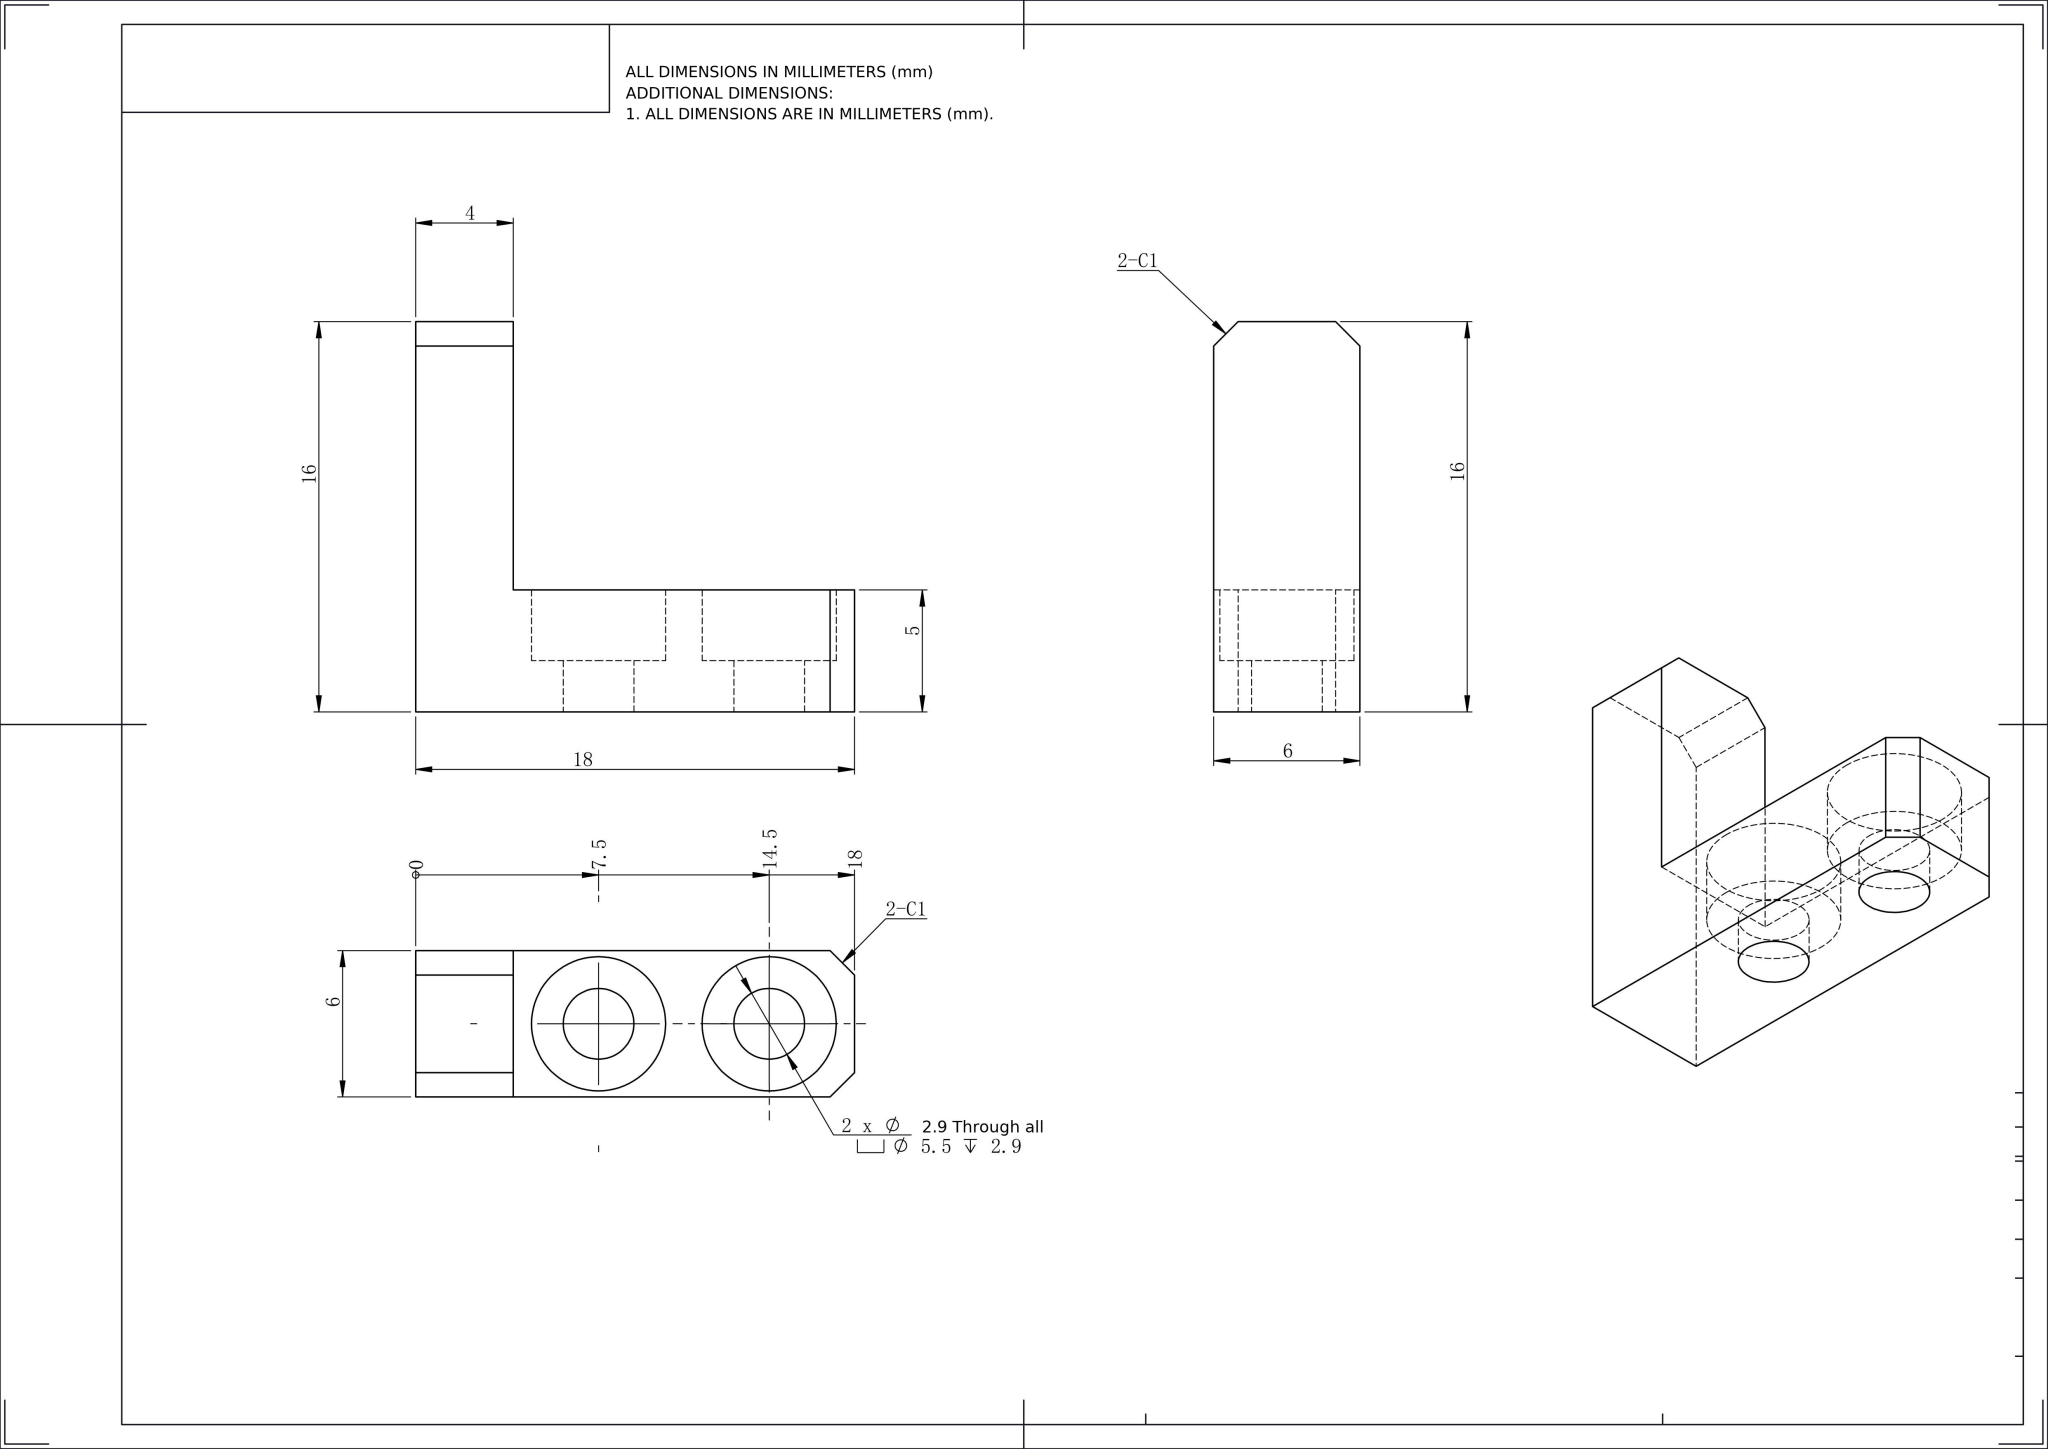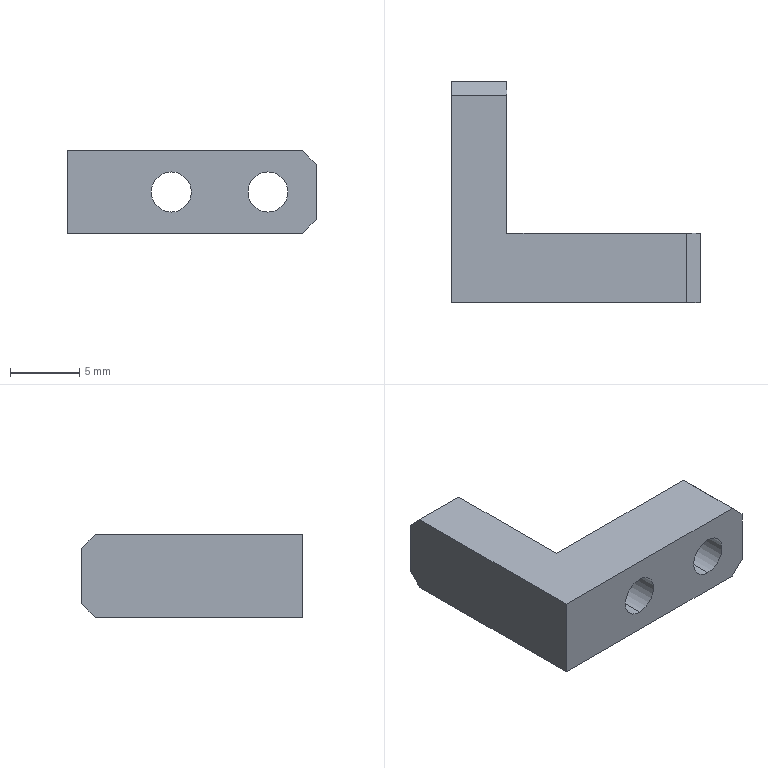Part | NX | mm | Chamfered Dual-Bore Clevis Block | 1 solid | 22 faces | box 18 x 16 x 6 mm | volume 629 mm3 | plane 14 | cylinder 8 | commonest cylinder face diameters 5.5 x4 2.9 x4
STEP:
#1=COLOUR_RGB('',0.7922,0.8196,0.9333);
#2=FILL_AREA_STYLE_COLOUR('',#1);
#3=FILL_AREA_STYLE('',(#2));
#4=SURFACE_STYLE_FILL_AREA(#3);
#5=SURFACE_SIDE_STYLE('',(#4));
#6=SURFACE_STYLE_USAGE(.BOTH.,#5);
#7=PRESENTATION_STYLE_ASSIGNMENT((#6));
#8=CARTESIAN_POINT('',(5.5,-5.9,-2.75));
#9=VERTEX_POINT('',#8);
#10=CARTESIAN_POINT('',(5.5,-5.9,2.75));
#11=VERTEX_POINT('',#10);
#12=CARTESIAN_POINT('',(5.5,-5.9,0.));
#13=DIRECTION('',(0.,1.,0.));
#14=DIRECTION('',(0.,0.,1.));
#15=AXIS2_PLACEMENT_3D('',#12,#13,#14);
#16=CIRCLE('',#15,2.75);
#17=EDGE_CURVE('',#9,#11,#16,.T.);
#18=ORIENTED_EDGE('',*,*,#17,.F.);
#19=CARTESIAN_POINT('',(5.5,-3.,-2.75));
#20=VERTEX_POINT('',#19);
#21=CARTESIAN_POINT('',(5.5,-3.,-2.75));
#22=DIRECTION('',(0.,1.,0.));
#23=VECTOR('',#22,1000.);
#24=LINE('',#21,#23);
#25=EDGE_CURVE('',#9,#20,#24,.T.);
#26=ORIENTED_EDGE('',*,*,#25,.T.);
#27=CARTESIAN_POINT('',(5.5,-3.,2.75));
#28=VERTEX_POINT('',#27);
#29=CARTESIAN_POINT('',(5.5,-3.,0.));
#30=DIRECTION('',(0.,1.,0.));
#31=DIRECTION('',(0.,0.,1.));
#32=AXIS2_PLACEMENT_3D('',#29,#30,#31);
#33=CIRCLE('',#32,2.75);
#34=EDGE_CURVE('',#20,#28,#33,.T.);
#35=ORIENTED_EDGE('',*,*,#34,.T.);
#36=CARTESIAN_POINT('',(5.5,-3.,2.75));
#37=DIRECTION('',(0.,1.,0.));
#38=VECTOR('',#37,1000.);
#39=LINE('',#36,#38);
#40=EDGE_CURVE('',#11,#28,#39,.T.);
#41=ORIENTED_EDGE('',*,*,#40,.F.);
#42=EDGE_LOOP('',(#18,#26,#35,#41));
#43=FACE_OUTER_BOUND('',#42,.T.);
#44=CARTESIAN_POINT('',(5.5,-3.,0.));
#45=DIRECTION('',(0.,1.,0.));
#46=DIRECTION('',(0.,0.,1.));
#47=AXIS2_PLACEMENT_3D('',#44,#45,#46);
#48=CYLINDRICAL_SURFACE('',#47,2.75);
#49=ADVANCED_FACE('',(#43),#48,.F.);
#50=CARTESIAN_POINT('',(5.5,-8.,-1.45));
#51=VERTEX_POINT('',#50);
#52=CARTESIAN_POINT('',(5.5,-8.,1.45));
#53=VERTEX_POINT('',#52);
#54=CARTESIAN_POINT('',(5.5,-8.,0.));
#55=DIRECTION('',(0.,1.,0.));
#56=DIRECTION('',(0.,0.,1.));
#57=AXIS2_PLACEMENT_3D('',#54,#55,#56);
#58=CIRCLE('',#57,1.45);
#59=EDGE_CURVE('',#51,#53,#58,.T.);
#60=ORIENTED_EDGE('',*,*,#59,.F.);
#61=CARTESIAN_POINT('',(5.5,-5.9,-1.45));
#62=VERTEX_POINT('',#61);
#63=CARTESIAN_POINT('',(5.5,-3.,-1.45));
#64=DIRECTION('',(0.,1.,0.));
#65=VECTOR('',#64,1000.);
#66=LINE('',#63,#65);
#67=EDGE_CURVE('',#51,#62,#66,.T.);
#68=ORIENTED_EDGE('',*,*,#67,.T.);
#69=CARTESIAN_POINT('',(5.5,-5.9,1.45));
#70=VERTEX_POINT('',#69);
#71=CARTESIAN_POINT('',(5.5,-5.9,0.));
#72=DIRECTION('',(0.,1.,0.));
#73=DIRECTION('',(0.,0.,1.));
#74=AXIS2_PLACEMENT_3D('',#71,#72,#73);
#75=CIRCLE('',#74,1.45);
#76=EDGE_CURVE('',#62,#70,#75,.T.);
#77=ORIENTED_EDGE('',*,*,#76,.T.);
#78=CARTESIAN_POINT('',(5.5,-3.,1.45));
#79=DIRECTION('',(0.,1.,0.));
#80=VECTOR('',#79,1000.);
#81=LINE('',#78,#80);
#82=EDGE_CURVE('',#53,#70,#81,.T.);
#83=ORIENTED_EDGE('',*,*,#82,.F.);
#84=EDGE_LOOP('',(#60,#68,#77,#83));
#85=FACE_OUTER_BOUND('',#84,.T.);
#86=CARTESIAN_POINT('',(5.5,-3.,0.));
#87=DIRECTION('',(0.,1.,0.));
#88=DIRECTION('',(0.,0.,1.));
#89=AXIS2_PLACEMENT_3D('',#86,#87,#88);
#90=CYLINDRICAL_SURFACE('',#89,1.45);
#91=ADVANCED_FACE('',(#85),#90,.F.);
#92=CARTESIAN_POINT('',(-1.5,-5.9,-2.75));
#93=VERTEX_POINT('',#92);
#94=CARTESIAN_POINT('',(-1.5,-5.9,2.75));
#95=VERTEX_POINT('',#94);
#96=CARTESIAN_POINT('',(-1.5,-5.9,0.));
#97=DIRECTION('',(0.,1.,0.));
#98=DIRECTION('',(0.,0.,1.));
#99=AXIS2_PLACEMENT_3D('',#96,#97,#98);
#100=CIRCLE('',#99,2.75);
#101=EDGE_CURVE('',#93,#95,#100,.T.);
#102=ORIENTED_EDGE('',*,*,#101,.F.);
#103=CARTESIAN_POINT('',(-1.5,-3.,-2.75));
#104=VERTEX_POINT('',#103);
#105=CARTESIAN_POINT('',(-1.5,-3.,-2.75));
#106=DIRECTION('',(0.,1.,0.));
#107=VECTOR('',#106,1000.);
#108=LINE('',#105,#107);
#109=EDGE_CURVE('',#93,#104,#108,.T.);
#110=ORIENTED_EDGE('',*,*,#109,.T.);
#111=CARTESIAN_POINT('',(-1.5,-3.,2.75));
#112=VERTEX_POINT('',#111);
#113=CARTESIAN_POINT('',(-1.5,-3.,0.));
#114=DIRECTION('',(0.,1.,0.));
#115=DIRECTION('',(0.,0.,1.));
#116=AXIS2_PLACEMENT_3D('',#113,#114,#115);
#117=CIRCLE('',#116,2.75);
#118=EDGE_CURVE('',#104,#112,#117,.T.);
#119=ORIENTED_EDGE('',*,*,#118,.T.);
#120=CARTESIAN_POINT('',(-1.5,-3.,2.75));
#121=DIRECTION('',(0.,1.,0.));
#122=VECTOR('',#121,1000.);
#123=LINE('',#120,#122);
#124=EDGE_CURVE('',#95,#112,#123,.T.);
#125=ORIENTED_EDGE('',*,*,#124,.F.);
#126=EDGE_LOOP('',(#102,#110,#119,#125));
#127=FACE_OUTER_BOUND('',#126,.T.);
#128=CARTESIAN_POINT('',(-1.5,-3.,0.));
#129=DIRECTION('',(0.,1.,0.));
#130=DIRECTION('',(0.,0.,1.));
#131=AXIS2_PLACEMENT_3D('',#128,#129,#130);
#132=CYLINDRICAL_SURFACE('',#131,2.75);
#133=ADVANCED_FACE('',(#127),#132,.F.);
#134=CARTESIAN_POINT('',(-1.5,-8.,-1.45));
#135=VERTEX_POINT('',#134);
#136=CARTESIAN_POINT('',(-1.5,-8.,1.45));
#137=VERTEX_POINT('',#136);
#138=CARTESIAN_POINT('',(-1.5,-8.,0.));
#139=DIRECTION('',(0.,1.,0.));
#140=DIRECTION('',(0.,0.,1.));
#141=AXIS2_PLACEMENT_3D('',#138,#139,#140);
#142=CIRCLE('',#141,1.45);
#143=EDGE_CURVE('',#135,#137,#142,.T.);
#144=ORIENTED_EDGE('',*,*,#143,.F.);
#145=CARTESIAN_POINT('',(-1.5,-5.9,-1.45));
#146=VERTEX_POINT('',#145);
#147=CARTESIAN_POINT('',(-1.5,-3.,-1.45));
#148=DIRECTION('',(0.,1.,0.));
#149=VECTOR('',#148,1000.);
#150=LINE('',#147,#149);
#151=EDGE_CURVE('',#135,#146,#150,.T.);
#152=ORIENTED_EDGE('',*,*,#151,.T.);
#153=CARTESIAN_POINT('',(-1.5,-5.9,1.45));
#154=VERTEX_POINT('',#153);
#155=CARTESIAN_POINT('',(-1.5,-5.9,0.));
#156=DIRECTION('',(0.,1.,0.));
#157=DIRECTION('',(0.,0.,1.));
#158=AXIS2_PLACEMENT_3D('',#155,#156,#157);
#159=CIRCLE('',#158,1.45);
#160=EDGE_CURVE('',#146,#154,#159,.T.);
#161=ORIENTED_EDGE('',*,*,#160,.T.);
#162=CARTESIAN_POINT('',(-1.5,-3.,1.45));
#163=DIRECTION('',(0.,1.,0.));
#164=VECTOR('',#163,1000.);
#165=LINE('',#162,#164);
#166=EDGE_CURVE('',#137,#154,#165,.T.);
#167=ORIENTED_EDGE('',*,*,#166,.F.);
#168=EDGE_LOOP('',(#144,#152,#161,#167));
#169=FACE_OUTER_BOUND('',#168,.T.);
#170=CARTESIAN_POINT('',(-1.5,-3.,0.));
#171=DIRECTION('',(0.,1.,0.));
#172=DIRECTION('',(0.,0.,1.));
#173=AXIS2_PLACEMENT_3D('',#170,#171,#172);
#174=CYLINDRICAL_SURFACE('',#173,1.45);
#175=ADVANCED_FACE('',(#169),#174,.F.);
#176=CARTESIAN_POINT('',(-9.,7.,3.));
#177=VERTEX_POINT('',#176);
#178=CARTESIAN_POINT('',(-9.,-8.,3.));
#179=VERTEX_POINT('',#178);
#180=CARTESIAN_POINT('',(-9.,-8.,3.));
#181=DIRECTION('',(0.,-1.,0.));
#182=VECTOR('',#181,1000.);
#183=LINE('',#180,#182);
#184=EDGE_CURVE('',#177,#179,#183,.T.);
#185=ORIENTED_EDGE('',*,*,#184,.F.);
#186=CARTESIAN_POINT('',(-9.,8.,2.));
#187=VERTEX_POINT('',#186);
#188=CARTESIAN_POINT('',(-9.,7.,3.));
#189=DIRECTION('',(0.,0.7071,-0.7071));
#190=VECTOR('',#189,1000.);
#191=LINE('',#188,#190);
#192=EDGE_CURVE('',#177,#187,#191,.T.);
#193=ORIENTED_EDGE('',*,*,#192,.T.);
#194=CARTESIAN_POINT('',(-9.,8.,-2.));
#195=VERTEX_POINT('',#194);
#196=CARTESIAN_POINT('',(-9.,8.,3.));
#197=DIRECTION('',(0.,0.,-1.));
#198=VECTOR('',#197,1000.);
#199=LINE('',#196,#198);
#200=EDGE_CURVE('',#187,#195,#199,.T.);
#201=ORIENTED_EDGE('',*,*,#200,.T.);
#202=CARTESIAN_POINT('',(-9.,7.,-3.));
#203=VERTEX_POINT('',#202);
#204=CARTESIAN_POINT('',(-9.,8.,-2.));
#205=DIRECTION('',(0.,-0.7071,-0.7071));
#206=VECTOR('',#205,1000.);
#207=LINE('',#204,#206);
#208=EDGE_CURVE('',#195,#203,#207,.T.);
#209=ORIENTED_EDGE('',*,*,#208,.T.);
#210=CARTESIAN_POINT('',(-9.,-8.,-3.));
#211=VERTEX_POINT('',#210);
#212=CARTESIAN_POINT('',(-9.,-8.,-3.));
#213=DIRECTION('',(0.,-1.,0.));
#214=VECTOR('',#213,1000.);
#215=LINE('',#212,#214);
#216=EDGE_CURVE('',#203,#211,#215,.T.);
#217=ORIENTED_EDGE('',*,*,#216,.T.);
#218=CARTESIAN_POINT('',(-9.,-8.,3.));
#219=DIRECTION('',(0.,0.,-1.));
#220=VECTOR('',#219,1000.);
#221=LINE('',#218,#220);
#222=EDGE_CURVE('',#179,#211,#221,.T.);
#223=ORIENTED_EDGE('',*,*,#222,.F.);
#224=EDGE_LOOP('',(#185,#193,#201,#209,#217,#223));
#225=FACE_OUTER_BOUND('',#224,.T.);
#226=CARTESIAN_POINT('',(-9.,-8.,3.));
#227=DIRECTION('',(1.,0.,0.));
#228=DIRECTION('',(0.,0.,-1.));
#229=AXIS2_PLACEMENT_3D('',#226,#227,#228);
#230=PLANE('',#229);
#231=ADVANCED_FACE('',(#225),#230,.F.);
#232=CARTESIAN_POINT('',(5.5,-8.,0.));
#233=DIRECTION('',(0.,1.,0.));
#234=DIRECTION('',(0.,0.,1.));
#235=AXIS2_PLACEMENT_3D('',#232,#233,#234);
#236=CIRCLE('',#235,1.45);
#237=EDGE_CURVE('',#53,#51,#236,.T.);
#238=ORIENTED_EDGE('',*,*,#237,.T.);
#239=ORIENTED_EDGE('',*,*,#59,.T.);
#240=EDGE_LOOP('',(#238,#239));
#241=FACE_BOUND('',#240,.T.);
#242=CARTESIAN_POINT('',(-1.5,-8.,0.));
#243=DIRECTION('',(0.,1.,0.));
#244=DIRECTION('',(0.,0.,1.));
#245=AXIS2_PLACEMENT_3D('',#242,#243,#244);
#246=CIRCLE('',#245,1.45);
#247=EDGE_CURVE('',#137,#135,#246,.T.);
#248=ORIENTED_EDGE('',*,*,#247,.T.);
#249=ORIENTED_EDGE('',*,*,#143,.T.);
#250=EDGE_LOOP('',(#248,#249));
#251=FACE_BOUND('',#250,.T.);
#252=CARTESIAN_POINT('',(8.,-8.,-3.));
#253=VERTEX_POINT('',#252);
#254=CARTESIAN_POINT('',(9.,-8.,-3.));
#255=DIRECTION('',(1.,0.,0.));
#256=VECTOR('',#255,1000.);
#257=LINE('',#254,#256);
#258=EDGE_CURVE('',#211,#253,#257,.T.);
#259=ORIENTED_EDGE('',*,*,#258,.T.);
#260=CARTESIAN_POINT('',(9.,-8.,-2.));
#261=VERTEX_POINT('',#260);
#262=CARTESIAN_POINT('',(9.,-8.,-2.));
#263=DIRECTION('',(0.7071,0.,0.7071));
#264=VECTOR('',#263,1000.);
#265=LINE('',#262,#264);
#266=EDGE_CURVE('',#253,#261,#265,.T.);
#267=ORIENTED_EDGE('',*,*,#266,.T.);
#268=CARTESIAN_POINT('',(9.,-8.,2.));
#269=VERTEX_POINT('',#268);
#270=CARTESIAN_POINT('',(9.,-8.,3.));
#271=DIRECTION('',(0.,0.,-1.));
#272=VECTOR('',#271,1000.);
#273=LINE('',#270,#272);
#274=EDGE_CURVE('',#269,#261,#273,.T.);
#275=ORIENTED_EDGE('',*,*,#274,.F.);
#276=CARTESIAN_POINT('',(8.,-8.,3.));
#277=VERTEX_POINT('',#276);
#278=CARTESIAN_POINT('',(8.,-8.,3.));
#279=DIRECTION('',(-0.7071,-0.,0.7071));
#280=VECTOR('',#279,1000.);
#281=LINE('',#278,#280);
#282=EDGE_CURVE('',#269,#277,#281,.T.);
#283=ORIENTED_EDGE('',*,*,#282,.T.);
#284=CARTESIAN_POINT('',(9.,-8.,3.));
#285=DIRECTION('',(1.,0.,0.));
#286=VECTOR('',#285,1000.);
#287=LINE('',#284,#286);
#288=EDGE_CURVE('',#179,#277,#287,.T.);
#289=ORIENTED_EDGE('',*,*,#288,.F.);
#290=ORIENTED_EDGE('',*,*,#222,.T.);
#291=EDGE_LOOP('',(#259,#267,#275,#283,#289,#290));
#292=FACE_OUTER_BOUND('',#291,.T.);
#293=CARTESIAN_POINT('',(9.,-8.,3.));
#294=DIRECTION('',(-0.,1.,0.));
#295=DIRECTION('',(-1.,-0.,0.));
#296=AXIS2_PLACEMENT_3D('',#293,#294,#295);
#297=PLANE('',#296);
#298=ADVANCED_FACE('',(#241,#251,#292),#297,.F.);
#299=ORIENTED_EDGE('',*,*,#274,.T.);
#300=CARTESIAN_POINT('',(9.,-3.,-2.));
#301=VERTEX_POINT('',#300);
#302=CARTESIAN_POINT('',(9.,-8.,-2.));
#303=DIRECTION('',(0.,1.,0.));
#304=VECTOR('',#303,1000.);
#305=LINE('',#302,#304);
#306=EDGE_CURVE('',#261,#301,#305,.T.);
#307=ORIENTED_EDGE('',*,*,#306,.T.);
#308=CARTESIAN_POINT('',(9.,-3.,2.));
#309=VERTEX_POINT('',#308);
#310=CARTESIAN_POINT('',(9.,-3.,3.));
#311=DIRECTION('',(0.,0.,-1.));
#312=VECTOR('',#311,1000.);
#313=LINE('',#310,#312);
#314=EDGE_CURVE('',#309,#301,#313,.T.);
#315=ORIENTED_EDGE('',*,*,#314,.F.);
#316=CARTESIAN_POINT('',(9.,-8.,2.));
#317=DIRECTION('',(0.,-1.,0.));
#318=VECTOR('',#317,1000.);
#319=LINE('',#316,#318);
#320=EDGE_CURVE('',#309,#269,#319,.T.);
#321=ORIENTED_EDGE('',*,*,#320,.T.);
#322=EDGE_LOOP('',(#299,#307,#315,#321));
#323=FACE_OUTER_BOUND('',#322,.T.);
#324=CARTESIAN_POINT('',(9.,-8.,3.));
#325=DIRECTION('',(-1.,0.,0.));
#326=DIRECTION('',(0.,0.,1.));
#327=AXIS2_PLACEMENT_3D('',#324,#325,#326);
#328=PLANE('',#327);
#329=ADVANCED_FACE('',(#323),#328,.F.);
#330=ORIENTED_EDGE('',*,*,#200,.F.);
#331=CARTESIAN_POINT('',(-5.,8.,2.));
#332=VERTEX_POINT('',#331);
#333=CARTESIAN_POINT('',(-5.,8.,2.));
#334=DIRECTION('',(1.,0.,0.));
#335=VECTOR('',#334,1000.);
#336=LINE('',#333,#335);
#337=EDGE_CURVE('',#187,#332,#336,.T.);
#338=ORIENTED_EDGE('',*,*,#337,.T.);
#339=CARTESIAN_POINT('',(-5.,8.,-2.));
#340=VERTEX_POINT('',#339);
#341=CARTESIAN_POINT('',(-5.,8.,3.));
#342=DIRECTION('',(0.,0.,-1.));
#343=VECTOR('',#342,1000.);
#344=LINE('',#341,#343);
#345=EDGE_CURVE('',#332,#340,#344,.T.);
#346=ORIENTED_EDGE('',*,*,#345,.T.);
#347=CARTESIAN_POINT('',(9.,8.,-2.));
#348=DIRECTION('',(-1.,-0.,0.));
#349=VECTOR('',#348,1000.);
#350=LINE('',#347,#349);
#351=EDGE_CURVE('',#340,#195,#350,.T.);
#352=ORIENTED_EDGE('',*,*,#351,.T.);
#353=EDGE_LOOP('',(#330,#338,#346,#352));
#354=FACE_OUTER_BOUND('',#353,.T.);
#355=CARTESIAN_POINT('',(9.,8.,3.));
#356=DIRECTION('',(0.,-1.,0.));
#357=DIRECTION('',(1.,0.,0.));
#358=AXIS2_PLACEMENT_3D('',#355,#356,#357);
#359=PLANE('',#358);
#360=ADVANCED_FACE('',(#354),#359,.F.);
#361=CARTESIAN_POINT('',(-5.,-3.,3.));
#362=VERTEX_POINT('',#361);
#363=CARTESIAN_POINT('',(-5.,7.,3.));
#364=VERTEX_POINT('',#363);
#365=CARTESIAN_POINT('',(-5.,8.,3.));
#366=DIRECTION('',(0.,1.,0.));
#367=VECTOR('',#366,1000.);
#368=LINE('',#365,#367);
#369=EDGE_CURVE('',#362,#364,#368,.T.);
#370=ORIENTED_EDGE('',*,*,#369,.T.);
#371=CARTESIAN_POINT('',(-9.,7.,3.));
#372=DIRECTION('',(-1.,-0.,0.));
#373=VECTOR('',#372,1000.);
#374=LINE('',#371,#373);
#375=EDGE_CURVE('',#364,#177,#374,.T.);
#376=ORIENTED_EDGE('',*,*,#375,.T.);
#377=ORIENTED_EDGE('',*,*,#184,.T.);
#378=ORIENTED_EDGE('',*,*,#288,.T.);
#379=CARTESIAN_POINT('',(8.,-3.,3.));
#380=VERTEX_POINT('',#379);
#381=CARTESIAN_POINT('',(8.,-3.,3.));
#382=DIRECTION('',(0.,1.,0.));
#383=VECTOR('',#382,1000.);
#384=LINE('',#381,#383);
#385=EDGE_CURVE('',#277,#380,#384,.T.);
#386=ORIENTED_EDGE('',*,*,#385,.T.);
#387=CARTESIAN_POINT('',(9.,-3.,3.));
#388=DIRECTION('',(-1.,0.,0.));
#389=VECTOR('',#388,1000.);
#390=LINE('',#387,#389);
#391=EDGE_CURVE('',#380,#362,#390,.T.);
#392=ORIENTED_EDGE('',*,*,#391,.T.);
#393=EDGE_LOOP('',(#370,#376,#377,#378,#386,#392));
#394=FACE_OUTER_BOUND('',#393,.T.);
#395=CARTESIAN_POINT('',(0.,0.,3.));
#396=DIRECTION('',(0.,0.,1.));
#397=DIRECTION('',(1.,0.,0.));
#398=AXIS2_PLACEMENT_3D('',#395,#396,#397);
#399=PLANE('',#398);
#400=ADVANCED_FACE('',(#394),#399,.T.);
#401=ORIENTED_EDGE('',*,*,#216,.F.);
#402=CARTESIAN_POINT('',(-5.,7.,-3.));
#403=VERTEX_POINT('',#402);
#404=CARTESIAN_POINT('',(-0.,7.,-3.));
#405=DIRECTION('',(1.,0.,0.));
#406=VECTOR('',#405,1000.);
#407=LINE('',#404,#406);
#408=EDGE_CURVE('',#203,#403,#407,.T.);
#409=ORIENTED_EDGE('',*,*,#408,.T.);
#410=CARTESIAN_POINT('',(-5.,-3.,-3.));
#411=VERTEX_POINT('',#410);
#412=CARTESIAN_POINT('',(-5.,8.,-3.));
#413=DIRECTION('',(0.,1.,0.));
#414=VECTOR('',#413,1000.);
#415=LINE('',#412,#414);
#416=EDGE_CURVE('',#411,#403,#415,.T.);
#417=ORIENTED_EDGE('',*,*,#416,.F.);
#418=CARTESIAN_POINT('',(8.,-3.,-3.));
#419=VERTEX_POINT('',#418);
#420=CARTESIAN_POINT('',(9.,-3.,-3.));
#421=DIRECTION('',(-1.,0.,0.));
#422=VECTOR('',#421,1000.);
#423=LINE('',#420,#422);
#424=EDGE_CURVE('',#419,#411,#423,.T.);
#425=ORIENTED_EDGE('',*,*,#424,.F.);
#426=CARTESIAN_POINT('',(8.,0.,-3.));
#427=DIRECTION('',(0.,-1.,0.));
#428=VECTOR('',#427,1000.);
#429=LINE('',#426,#428);
#430=EDGE_CURVE('',#419,#253,#429,.T.);
#431=ORIENTED_EDGE('',*,*,#430,.T.);
#432=ORIENTED_EDGE('',*,*,#258,.F.);
#433=EDGE_LOOP('',(#401,#409,#417,#425,#431,#432));
#434=FACE_OUTER_BOUND('',#433,.T.);
#435=CARTESIAN_POINT('',(0.,0.,-3.));
#436=DIRECTION('',(0.,0.,1.));
#437=DIRECTION('',(1.,0.,0.));
#438=AXIS2_PLACEMENT_3D('',#435,#436,#437);
#439=PLANE('',#438);
#440=ADVANCED_FACE('',(#434),#439,.F.);
#441=ORIENTED_EDGE('',*,*,#345,.F.);
#442=CARTESIAN_POINT('',(-5.,7.,3.));
#443=DIRECTION('',(-0.,-0.7071,0.7071));
#444=VECTOR('',#443,1000.);
#445=LINE('',#442,#444);
#446=EDGE_CURVE('',#332,#364,#445,.T.);
#447=ORIENTED_EDGE('',*,*,#446,.T.);
#448=ORIENTED_EDGE('',*,*,#369,.F.);
#449=CARTESIAN_POINT('',(-5.,-3.,3.));
#450=DIRECTION('',(0.,0.,-1.));
#451=VECTOR('',#450,1000.);
#452=LINE('',#449,#451);
#453=EDGE_CURVE('',#362,#411,#452,.T.);
#454=ORIENTED_EDGE('',*,*,#453,.T.);
#455=ORIENTED_EDGE('',*,*,#416,.T.);
#456=CARTESIAN_POINT('',(-5.,8.,-2.));
#457=DIRECTION('',(0.,0.7071,0.7071));
#458=VECTOR('',#457,1000.);
#459=LINE('',#456,#458);
#460=EDGE_CURVE('',#403,#340,#459,.T.);
#461=ORIENTED_EDGE('',*,*,#460,.T.);
#462=EDGE_LOOP('',(#441,#447,#448,#454,#455,#461));
#463=FACE_OUTER_BOUND('',#462,.T.);
#464=CARTESIAN_POINT('',(-5.,8.,3.));
#465=DIRECTION('',(-1.,0.,0.));
#466=DIRECTION('',(-0.,-1.,0.));
#467=AXIS2_PLACEMENT_3D('',#464,#465,#466);
#468=PLANE('',#467);
#469=ADVANCED_FACE('',(#463),#468,.F.);
#470=CARTESIAN_POINT('',(5.5,-3.,0.));
#471=DIRECTION('',(0.,1.,0.));
#472=DIRECTION('',(0.,0.,1.));
#473=AXIS2_PLACEMENT_3D('',#470,#471,#472);
#474=CIRCLE('',#473,2.75);
#475=EDGE_CURVE('',#28,#20,#474,.T.);
#476=ORIENTED_EDGE('',*,*,#475,.F.);
#477=ORIENTED_EDGE('',*,*,#34,.F.);
#478=EDGE_LOOP('',(#476,#477));
#479=FACE_BOUND('',#478,.T.);
#480=CARTESIAN_POINT('',(-1.5,-3.,0.));
#481=DIRECTION('',(0.,1.,0.));
#482=DIRECTION('',(0.,0.,1.));
#483=AXIS2_PLACEMENT_3D('',#480,#481,#482);
#484=CIRCLE('',#483,2.75);
#485=EDGE_CURVE('',#112,#104,#484,.T.);
#486=ORIENTED_EDGE('',*,*,#485,.F.);
#487=ORIENTED_EDGE('',*,*,#118,.F.);
#488=EDGE_LOOP('',(#486,#487));
#489=FACE_BOUND('',#488,.T.);
#490=ORIENTED_EDGE('',*,*,#314,.T.);
#491=CARTESIAN_POINT('',(9.,-3.,-2.));
#492=DIRECTION('',(-0.7071,0.,-0.7071));
#493=VECTOR('',#492,1000.);
#494=LINE('',#491,#493);
#495=EDGE_CURVE('',#301,#419,#494,.T.);
#496=ORIENTED_EDGE('',*,*,#495,.T.);
#497=ORIENTED_EDGE('',*,*,#424,.T.);
#498=ORIENTED_EDGE('',*,*,#453,.F.);
#499=ORIENTED_EDGE('',*,*,#391,.F.);
#500=CARTESIAN_POINT('',(8.,-3.,3.));
#501=DIRECTION('',(0.7071,-0.,-0.7071));
#502=VECTOR('',#501,1000.);
#503=LINE('',#500,#502);
#504=EDGE_CURVE('',#380,#309,#503,.T.);
#505=ORIENTED_EDGE('',*,*,#504,.T.);
#506=EDGE_LOOP('',(#490,#496,#497,#498,#499,#505));
#507=FACE_OUTER_BOUND('',#506,.T.);
#508=CARTESIAN_POINT('',(9.,-3.,3.));
#509=DIRECTION('',(-0.,-1.,0.));
#510=DIRECTION('',(1.,-0.,0.));
#511=AXIS2_PLACEMENT_3D('',#508,#509,#510);
#512=PLANE('',#511);
#513=ADVANCED_FACE('',(#479,#489,#507),#512,.F.);
#514=ORIENTED_EDGE('',*,*,#151,.F.);
#515=ORIENTED_EDGE('',*,*,#247,.F.);
#516=ORIENTED_EDGE('',*,*,#166,.T.);
#517=CARTESIAN_POINT('',(-1.5,-5.9,0.));
#518=DIRECTION('',(0.,1.,0.));
#519=DIRECTION('',(0.,0.,1.));
#520=AXIS2_PLACEMENT_3D('',#517,#518,#519);
#521=CIRCLE('',#520,1.45);
#522=EDGE_CURVE('',#154,#146,#521,.T.);
#523=ORIENTED_EDGE('',*,*,#522,.T.);
#524=EDGE_LOOP('',(#514,#515,#516,#523));
#525=FACE_OUTER_BOUND('',#524,.T.);
#526=CARTESIAN_POINT('',(-1.5,-3.,0.));
#527=DIRECTION('',(0.,1.,0.));
#528=DIRECTION('',(0.,0.,1.));
#529=AXIS2_PLACEMENT_3D('',#526,#527,#528);
#530=CYLINDRICAL_SURFACE('',#529,1.45);
#531=ADVANCED_FACE('',(#525),#530,.F.);
#532=ORIENTED_EDGE('',*,*,#522,.F.);
#533=ORIENTED_EDGE('',*,*,#160,.F.);
#534=EDGE_LOOP('',(#532,#533));
#535=FACE_BOUND('',#534,.T.);
#536=CARTESIAN_POINT('',(-1.5,-5.9,0.));
#537=DIRECTION('',(0.,1.,0.));
#538=DIRECTION('',(0.,0.,1.));
#539=AXIS2_PLACEMENT_3D('',#536,#537,#538);
#540=CIRCLE('',#539,2.75);
#541=EDGE_CURVE('',#95,#93,#540,.T.);
#542=ORIENTED_EDGE('',*,*,#541,.T.);
#543=ORIENTED_EDGE('',*,*,#101,.T.);
#544=EDGE_LOOP('',(#542,#543));
#545=FACE_OUTER_BOUND('',#544,.T.);
#546=CARTESIAN_POINT('',(-0.05,-5.9,0.));
#547=DIRECTION('',(0.,-1.,0.));
#548=DIRECTION('',(0.,0.,-1.));
#549=AXIS2_PLACEMENT_3D('',#546,#547,#548);
#550=PLANE('',#549);
#551=ADVANCED_FACE('',(#535,#545),#550,.F.);
#552=ORIENTED_EDGE('',*,*,#109,.F.);
#553=ORIENTED_EDGE('',*,*,#541,.F.);
#554=ORIENTED_EDGE('',*,*,#124,.T.);
#555=ORIENTED_EDGE('',*,*,#485,.T.);
#556=EDGE_LOOP('',(#552,#553,#554,#555));
#557=FACE_OUTER_BOUND('',#556,.T.);
#558=CARTESIAN_POINT('',(-1.5,-3.,0.));
#559=DIRECTION('',(0.,1.,0.));
#560=DIRECTION('',(0.,0.,1.));
#561=AXIS2_PLACEMENT_3D('',#558,#559,#560);
#562=CYLINDRICAL_SURFACE('',#561,2.75);
#563=ADVANCED_FACE('',(#557),#562,.F.);
#564=ORIENTED_EDGE('',*,*,#67,.F.);
#565=ORIENTED_EDGE('',*,*,#237,.F.);
#566=ORIENTED_EDGE('',*,*,#82,.T.);
#567=CARTESIAN_POINT('',(5.5,-5.9,0.));
#568=DIRECTION('',(0.,1.,0.));
#569=DIRECTION('',(0.,0.,1.));
#570=AXIS2_PLACEMENT_3D('',#567,#568,#569);
#571=CIRCLE('',#570,1.45);
#572=EDGE_CURVE('',#70,#62,#571,.T.);
#573=ORIENTED_EDGE('',*,*,#572,.T.);
#574=EDGE_LOOP('',(#564,#565,#566,#573));
#575=FACE_OUTER_BOUND('',#574,.T.);
#576=CARTESIAN_POINT('',(5.5,-3.,0.));
#577=DIRECTION('',(0.,1.,0.));
#578=DIRECTION('',(0.,0.,1.));
#579=AXIS2_PLACEMENT_3D('',#576,#577,#578);
#580=CYLINDRICAL_SURFACE('',#579,1.45);
#581=ADVANCED_FACE('',(#575),#580,.F.);
#582=ORIENTED_EDGE('',*,*,#572,.F.);
#583=ORIENTED_EDGE('',*,*,#76,.F.);
#584=EDGE_LOOP('',(#582,#583));
#585=FACE_BOUND('',#584,.T.);
#586=CARTESIAN_POINT('',(5.5,-5.9,0.));
#587=DIRECTION('',(0.,1.,0.));
#588=DIRECTION('',(0.,0.,1.));
#589=AXIS2_PLACEMENT_3D('',#586,#587,#588);
#590=CIRCLE('',#589,2.75);
#591=EDGE_CURVE('',#11,#9,#590,.T.);
#592=ORIENTED_EDGE('',*,*,#591,.T.);
#593=ORIENTED_EDGE('',*,*,#17,.T.);
#594=EDGE_LOOP('',(#592,#593));
#595=FACE_OUTER_BOUND('',#594,.T.);
#596=CARTESIAN_POINT('',(6.95,-5.9,0.));
#597=DIRECTION('',(0.,-1.,0.));
#598=DIRECTION('',(0.,0.,-1.));
#599=AXIS2_PLACEMENT_3D('',#596,#597,#598);
#600=PLANE('',#599);
#601=ADVANCED_FACE('',(#585,#595),#600,.F.);
#602=ORIENTED_EDGE('',*,*,#25,.F.);
#603=ORIENTED_EDGE('',*,*,#591,.F.);
#604=ORIENTED_EDGE('',*,*,#40,.T.);
#605=ORIENTED_EDGE('',*,*,#475,.T.);
#606=EDGE_LOOP('',(#602,#603,#604,#605));
#607=FACE_OUTER_BOUND('',#606,.T.);
#608=CARTESIAN_POINT('',(5.5,-3.,0.));
#609=DIRECTION('',(0.,1.,0.));
#610=DIRECTION('',(0.,0.,1.));
#611=AXIS2_PLACEMENT_3D('',#608,#609,#610);
#612=CYLINDRICAL_SURFACE('',#611,2.75);
#613=ADVANCED_FACE('',(#607),#612,.F.);
#614=ORIENTED_EDGE('',*,*,#446,.F.);
#615=ORIENTED_EDGE('',*,*,#337,.F.);
#616=ORIENTED_EDGE('',*,*,#192,.F.);
#617=ORIENTED_EDGE('',*,*,#375,.F.);
#618=EDGE_LOOP('',(#614,#615,#616,#617));
#619=FACE_OUTER_BOUND('',#618,.T.);
#620=CARTESIAN_POINT('',(-0.,7.,3.));
#621=DIRECTION('',(-0.,0.7071,0.7071));
#622=DIRECTION('',(1.,0.,0.));
#623=AXIS2_PLACEMENT_3D('',#620,#621,#622);
#624=PLANE('',#623);
#625=ADVANCED_FACE('',(#619),#624,.T.);
#626=ORIENTED_EDGE('',*,*,#460,.F.);
#627=ORIENTED_EDGE('',*,*,#408,.F.);
#628=ORIENTED_EDGE('',*,*,#208,.F.);
#629=ORIENTED_EDGE('',*,*,#351,.F.);
#630=EDGE_LOOP('',(#626,#627,#628,#629));
#631=FACE_OUTER_BOUND('',#630,.T.);
#632=CARTESIAN_POINT('',(9.,8.,-2.));
#633=DIRECTION('',(0.,-0.7071,0.7071));
#634=DIRECTION('',(-1.,-0.,0.));
#635=AXIS2_PLACEMENT_3D('',#632,#633,#634);
#636=PLANE('',#635);
#637=ADVANCED_FACE('',(#631),#636,.F.);
#638=ORIENTED_EDGE('',*,*,#266,.F.);
#639=ORIENTED_EDGE('',*,*,#430,.F.);
#640=ORIENTED_EDGE('',*,*,#495,.F.);
#641=ORIENTED_EDGE('',*,*,#306,.F.);
#642=EDGE_LOOP('',(#638,#639,#640,#641));
#643=FACE_OUTER_BOUND('',#642,.T.);
#644=CARTESIAN_POINT('',(9.,-8.,-2.));
#645=DIRECTION('',(-0.7071,0.,0.7071));
#646=DIRECTION('',(0.,1.,0.));
#647=AXIS2_PLACEMENT_3D('',#644,#645,#646);
#648=PLANE('',#647);
#649=ADVANCED_FACE('',(#643),#648,.F.);
#650=ORIENTED_EDGE('',*,*,#282,.F.);
#651=ORIENTED_EDGE('',*,*,#320,.F.);
#652=ORIENTED_EDGE('',*,*,#504,.F.);
#653=ORIENTED_EDGE('',*,*,#385,.F.);
#654=EDGE_LOOP('',(#650,#651,#652,#653));
#655=FACE_OUTER_BOUND('',#654,.T.);
#656=CARTESIAN_POINT('',(8.,0.,3.));
#657=DIRECTION('',(0.7071,0.,0.7071));
#658=DIRECTION('',(0.,-1.,0.));
#659=AXIS2_PLACEMENT_3D('',#656,#657,#658);
#660=PLANE('',#659);
#661=ADVANCED_FACE('',(#655),#660,.T.);
#662=CLOSED_SHELL('',(#49,#91,#133,#175,#231,#298,#329,#360,#400,#440,#469,#513,#531,#551,#563,#581,#601,#613,#625,#637,#649,#661));
#663=MANIFOLD_SOLID_BREP('',#662);
#664=STYLED_ITEM('',(#7),#663);
#665=PRESENTATION_LAYER_ASSIGNMENT('','',(#664));
#666=CARTESIAN_POINT('',(0.,0.,0.));
#667=DIRECTION('',(0.,0.,1.));
#668=DIRECTION('',(1.,0.,0.));
#669=AXIS2_PLACEMENT_3D('',#666,#667,#668);
#670=(LENGTH_UNIT()NAMED_UNIT(*)SI_UNIT(.MILLI.,.METRE.));
#671=UNCERTAINTY_MEASURE_WITH_UNIT(LENGTH_MEASURE(0.00001),#670,'','');
#672=(NAMED_UNIT(*)PLANE_ANGLE_UNIT()SI_UNIT($,.RADIAN.));
#673=(NAMED_UNIT(*)SI_UNIT($,.STERADIAN.)SOLID_ANGLE_UNIT());
#674=(GEOMETRIC_REPRESENTATION_CONTEXT(3)GLOBAL_UNCERTAINTY_ASSIGNED_CONTEXT((#671))GLOBAL_UNIT_ASSIGNED_CONTEXT((#670,#672,#673))REPRESENTATION_CONTEXT('',''));
#675=ADVANCED_BREP_SHAPE_REPRESENTATION('',(#663,#669),#674);
#676=(LENGTH_UNIT()NAMED_UNIT(*)SI_UNIT(.MILLI.,.METRE.));
#677=UNCERTAINTY_MEASURE_WITH_UNIT(LENGTH_MEASURE(0.00001),#676,'','');
#678=(NAMED_UNIT(*)PLANE_ANGLE_UNIT()SI_UNIT($,.RADIAN.));
#679=(NAMED_UNIT(*)SI_UNIT($,.STERADIAN.)SOLID_ANGLE_UNIT());
#680=(GEOMETRIC_REPRESENTATION_CONTEXT(3)GLOBAL_UNCERTAINTY_ASSIGNED_CONTEXT((#677))GLOBAL_UNIT_ASSIGNED_CONTEXT((#676,#678,#679))REPRESENTATION_CONTEXT('',''));
#681=MECHANICAL_DESIGN_GEOMETRIC_PRESENTATION_REPRESENTATION('',(#664),#680);